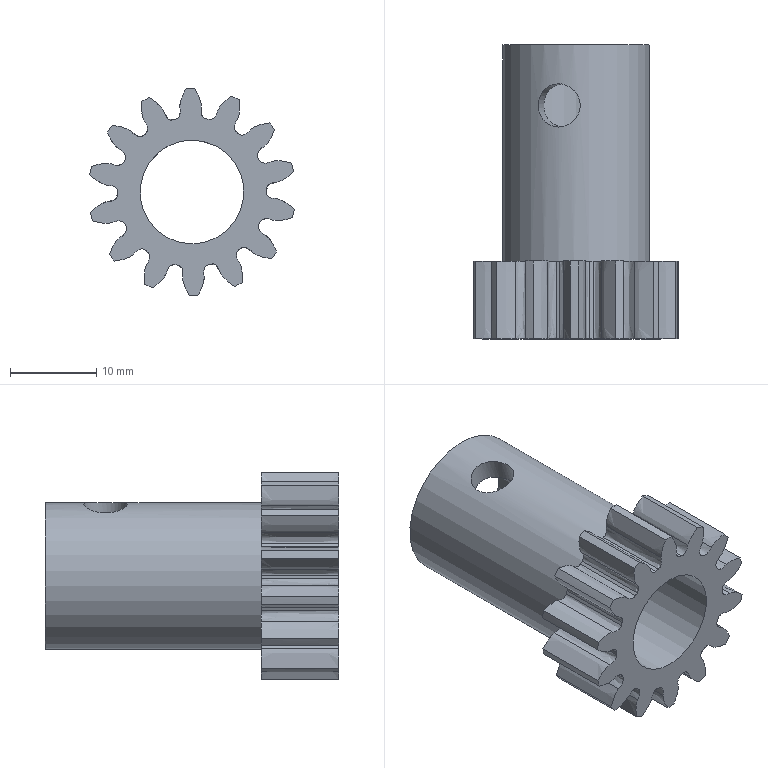Component | NX | GEAR_SHAFT | 1 solid | 90 faces | volume 4809 mm3 | other 70 | cylinder 17 | plane 3 | commonest cylinder face diameters 17.25 x14 17 x1 12 x1 5 x1